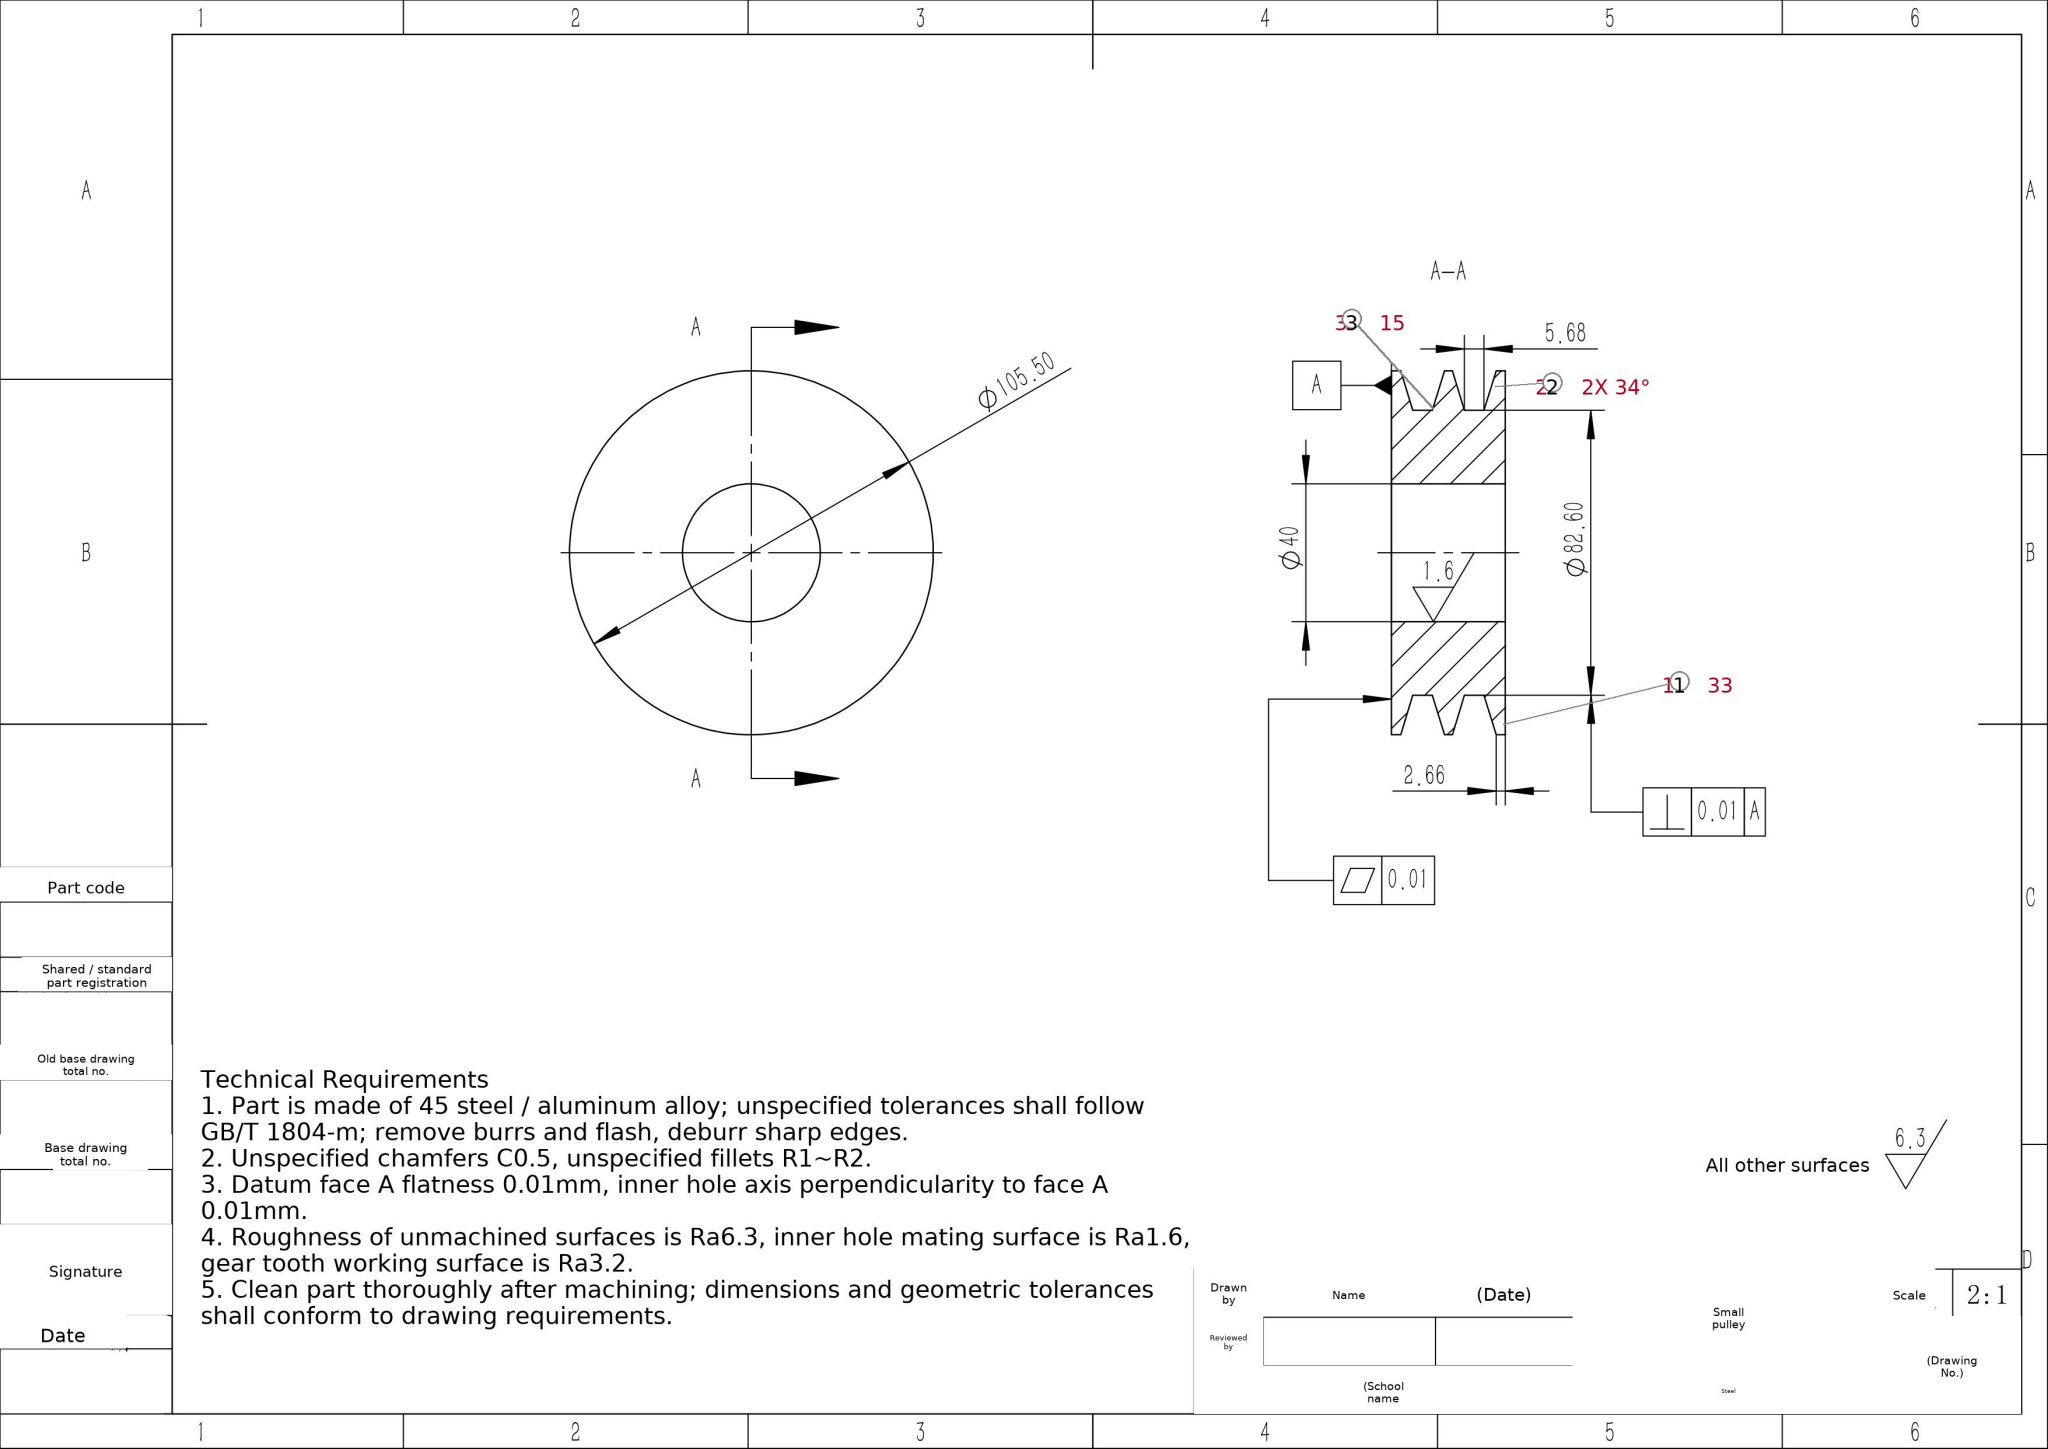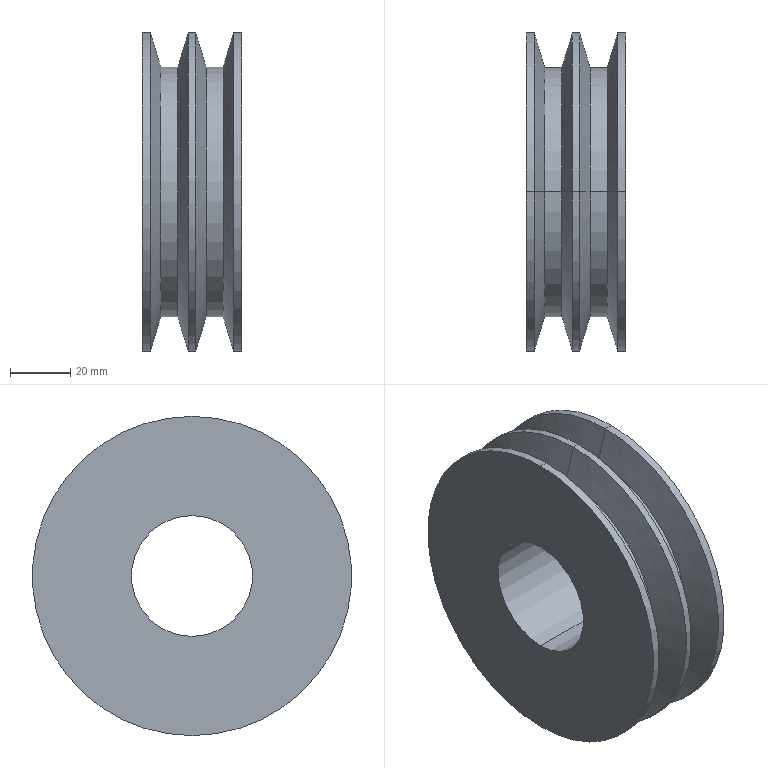Part | SolidWorks | mm | material 45 steel / aluminum alloy | 1 solid | 22 faces | box 33 x 105.5 x 105.5 mm | volume 183925 mm3 | cylinder 12 | cone 8 | plane 2 | commonest cylinder face diameters 105.5 x6 82.6 x4 40 x2
build123d program:
from build123d import *

# Parameters (mm, degrees)
LPATTERN1_COUNT         = 2
LPATTERN1_PITCH         = 15
CHAMFER1_SIZE           = 1
SKETCH4_W               = 5
SKETCH4_H               = 2.3
CUT_EXTRUDE1_DEPTH      = 82.573
CUT_EXTRUDE2_DEPTH      = 82.173
CUT_EXTRUDE2_DEPTH_BACK = 82.173
SKETCH5_R               = 20


with BuildPart() as part:
    # Sketch1 → Revolve1 (revolve)
    with BuildSketch(Plane.XY, mode=Mode.PRIVATE) as revolve1_sk:
        Polygon((0, 8), (0, 52.75), (33, 52.75), (33, 16), (32, 16), (32, 8), align=None)
    revolve(revolve1_sk.sketch.rotate(Axis((0, 0, 0), (1, 0, 0)), 90), axis=Axis((0, 0, 0), (1, 0, 0)))

    # Sketch2 → Cut-Revolve1 (revolve, cut)
    with BuildSketch(Plane.XY, mode=Mode.PRIVATE) as cut_revolve1_sk:
        Polygon((11.84, 41.3), (15.341, 52.75), (2.659, 52.75), (6.16, 41.3), align=None)
    cut_revolve1 = revolve(cut_revolve1_sk.sketch.rotate(Axis((0, 0, 0), (1, 0, 0)), 90), axis=Axis((0, 0, 0), (1, 0, 0)), mode=Mode.SUBTRACT)

    # LPattern1: Cut-Revolve1 ×2
    with Locations(*[(i * LPATTERN1_PITCH, 0, 0) for i in range(1, LPATTERN1_COUNT)]):
        add(cut_revolve1, mode=Mode.SUBTRACT)

    # Chamfer1
    chamfer1_edges = [part.edges().sort_by_distance(p)[0] for p in [
        (0, 0, -8),
        (32, 0, -8),
    ]]
    chamfer(chamfer1_edges, length=CHAMFER1_SIZE)

    # Sketch4 → Cut-Extrude1 (cut, through all)
    with BuildSketch(Plane.ZY):
        with Locations((0, 8.749)):
            Rectangle(SKETCH4_W, SKETCH4_H)
    extrude(amount=-CUT_EXTRUDE1_DEPTH, mode=Mode.SUBTRACT)

    # Sketch5 → Cut-Extrude2 (cut, two sides: drawn at the far end of the back side and taken through both)
    with BuildSketch(Plane(origin=(32, 0, 0), x_dir=(0, 0, -1), z_dir=(1, 0, 0)).offset(-CUT_EXTRUDE2_DEPTH_BACK)):
        Circle(SKETCH5_R)
    extrude(amount=CUT_EXTRUDE2_DEPTH + CUT_EXTRUDE2_DEPTH_BACK, mode=Mode.SUBTRACT)


solid = part.part
STEP:
#1=CARTESIAN_POINT('',(0.,0.,20.));
#2=VERTEX_POINT('',#1);
#3=CARTESIAN_POINT('',(0.,0.,-20.));
#4=VERTEX_POINT('',#3);
#5=CARTESIAN_POINT('',(0.,0.,0.));
#6=DIRECTION('',(1.,0.,0.));
#7=DIRECTION('',(0.,0.,-1.));
#8=AXIS2_PLACEMENT_3D('',#5,#6,#7);
#9=CIRCLE('',#8,20.);
#10=EDGE_CURVE('',#2,#4,#9,.T.);
#11=ORIENTED_EDGE('',*,*,#10,.F.);
#12=CARTESIAN_POINT('',(33.,0.,20.));
#13=VERTEX_POINT('',#12);
#14=CARTESIAN_POINT('',(0.,0.,20.));
#15=DIRECTION('',(1.,0.,0.));
#16=VECTOR('',#15,1000.);
#17=LINE('',#14,#16);
#18=EDGE_CURVE('',#2,#13,#17,.T.);
#19=ORIENTED_EDGE('',*,*,#18,.T.);
#20=CARTESIAN_POINT('',(33.,0.,-20.));
#21=VERTEX_POINT('',#20);
#22=CARTESIAN_POINT('',(33.,0.,0.));
#23=DIRECTION('',(1.,0.,0.));
#24=DIRECTION('',(0.,0.,-1.));
#25=AXIS2_PLACEMENT_3D('',#22,#23,#24);
#26=CIRCLE('',#25,20.);
#27=EDGE_CURVE('',#13,#21,#26,.T.);
#28=ORIENTED_EDGE('',*,*,#27,.T.);
#29=CARTESIAN_POINT('',(0.,0.,-20.));
#30=DIRECTION('',(1.,0.,0.));
#31=VECTOR('',#30,1000.);
#32=LINE('',#29,#31);
#33=EDGE_CURVE('',#4,#21,#32,.T.);
#34=ORIENTED_EDGE('',*,*,#33,.F.);
#35=EDGE_LOOP('',(#11,#19,#28,#34));
#36=FACE_OUTER_BOUND('',#35,.T.);
#37=CARTESIAN_POINT('',(0.,0.,0.));
#38=DIRECTION('',(1.,0.,0.));
#39=DIRECTION('',(0.,0.,-1.));
#40=AXIS2_PLACEMENT_3D('',#37,#38,#39);
#41=CYLINDRICAL_SURFACE('',#40,20.);
#42=ADVANCED_FACE('',(#36),#41,.F.);
#43=CARTESIAN_POINT('',(21.16,0.,41.3));
#44=VERTEX_POINT('',#43);
#45=CARTESIAN_POINT('',(21.16,0.,-41.3));
#46=VERTEX_POINT('',#45);
#47=CARTESIAN_POINT('',(21.16,0.,0.));
#48=DIRECTION('',(-1.,0.,0.));
#49=DIRECTION('',(0.,0.,1.));
#50=AXIS2_PLACEMENT_3D('',#47,#48,#49);
#51=CIRCLE('',#50,41.3);
#52=EDGE_CURVE('',#44,#46,#51,.T.);
#53=ORIENTED_EDGE('',*,*,#52,.T.);
#54=CARTESIAN_POINT('',(17.659,0.,-52.75));
#55=VERTEX_POINT('',#54);
#56=CARTESIAN_POINT('',(17.659,0.,-52.75));
#57=DIRECTION('',(-0.2924,0.,-0.9563));
#58=VECTOR('',#57,1000.);
#59=LINE('',#56,#58);
#60=EDGE_CURVE('',#46,#55,#59,.T.);
#61=ORIENTED_EDGE('',*,*,#60,.T.);
#62=CARTESIAN_POINT('',(17.659,0.,52.75));
#63=VERTEX_POINT('',#62);
#64=CARTESIAN_POINT('',(17.659,0.,0.));
#65=DIRECTION('',(-1.,0.,0.));
#66=DIRECTION('',(0.,0.,1.));
#67=AXIS2_PLACEMENT_3D('',#64,#65,#66);
#68=CIRCLE('',#67,52.75);
#69=EDGE_CURVE('',#63,#55,#68,.T.);
#70=ORIENTED_EDGE('',*,*,#69,.F.);
#71=CARTESIAN_POINT('',(17.659,0.,52.75));
#72=DIRECTION('',(-0.2924,0.,0.9563));
#73=VECTOR('',#72,1000.);
#74=LINE('',#71,#73);
#75=EDGE_CURVE('',#44,#63,#74,.T.);
#76=ORIENTED_EDGE('',*,*,#75,.F.);
#77=EDGE_LOOP('',(#53,#61,#70,#76));
#78=FACE_OUTER_BOUND('',#77,.T.);
#79=CARTESIAN_POINT('',(17.659,0.,0.));
#80=DIRECTION('',(-1.,0.,0.));
#81=DIRECTION('',(0.,0.,1.));
#82=AXIS2_PLACEMENT_3D('',#79,#80,#81);
#83=CONICAL_SURFACE('',#82,52.75,1.274);
#84=ADVANCED_FACE('',(#78),#83,.T.);
#85=CARTESIAN_POINT('',(26.84,0.,41.3));
#86=VERTEX_POINT('',#85);
#87=CARTESIAN_POINT('',(26.84,0.,-41.3));
#88=VERTEX_POINT('',#87);
#89=CARTESIAN_POINT('',(26.84,0.,0.));
#90=DIRECTION('',(-1.,0.,0.));
#91=DIRECTION('',(0.,0.,1.));
#92=AXIS2_PLACEMENT_3D('',#89,#90,#91);
#93=CIRCLE('',#92,41.3);
#94=EDGE_CURVE('',#86,#88,#93,.T.);
#95=ORIENTED_EDGE('',*,*,#94,.F.);
#96=CARTESIAN_POINT('',(30.341,0.,52.75));
#97=VERTEX_POINT('',#96);
#98=CARTESIAN_POINT('',(26.84,0.,41.3));
#99=DIRECTION('',(0.2924,0.,0.9563));
#100=VECTOR('',#99,1000.);
#101=LINE('',#98,#100);
#102=EDGE_CURVE('',#86,#97,#101,.T.);
#103=ORIENTED_EDGE('',*,*,#102,.T.);
#104=CARTESIAN_POINT('',(30.341,0.,-52.75));
#105=VERTEX_POINT('',#104);
#106=CARTESIAN_POINT('',(30.341,0.,0.));
#107=DIRECTION('',(-1.,0.,0.));
#108=DIRECTION('',(0.,0.,1.));
#109=AXIS2_PLACEMENT_3D('',#106,#107,#108);
#110=CIRCLE('',#109,52.75);
#111=EDGE_CURVE('',#97,#105,#110,.T.);
#112=ORIENTED_EDGE('',*,*,#111,.T.);
#113=CARTESIAN_POINT('',(26.84,0.,-41.3));
#114=DIRECTION('',(0.2924,0.,-0.9563));
#115=VECTOR('',#114,1000.);
#116=LINE('',#113,#115);
#117=EDGE_CURVE('',#88,#105,#116,.T.);
#118=ORIENTED_EDGE('',*,*,#117,.F.);
#119=EDGE_LOOP('',(#95,#103,#112,#118));
#120=FACE_OUTER_BOUND('',#119,.T.);
#121=CARTESIAN_POINT('',(26.84,0.,0.));
#122=DIRECTION('',(1.,0.,0.));
#123=DIRECTION('',(0.,0.,-1.));
#124=AXIS2_PLACEMENT_3D('',#121,#122,#123);
#125=CONICAL_SURFACE('',#124,41.3,1.274);
#126=ADVANCED_FACE('',(#120),#125,.T.);
#127=ORIENTED_EDGE('',*,*,#94,.T.);
#128=CARTESIAN_POINT('',(15.,0.,-41.3));
#129=DIRECTION('',(-1.,0.,0.));
#130=VECTOR('',#129,1000.);
#131=LINE('',#128,#130);
#132=EDGE_CURVE('',#88,#46,#131,.T.);
#133=ORIENTED_EDGE('',*,*,#132,.T.);
#134=ORIENTED_EDGE('',*,*,#52,.F.);
#135=CARTESIAN_POINT('',(15.,0.,41.3));
#136=DIRECTION('',(-1.,0.,0.));
#137=VECTOR('',#136,1000.);
#138=LINE('',#135,#137);
#139=EDGE_CURVE('',#86,#44,#138,.T.);
#140=ORIENTED_EDGE('',*,*,#139,.F.);
#141=EDGE_LOOP('',(#127,#133,#134,#140));
#142=FACE_OUTER_BOUND('',#141,.T.);
#143=CARTESIAN_POINT('',(15.,0.,0.));
#144=DIRECTION('',(-1.,0.,0.));
#145=DIRECTION('',(0.,0.,1.));
#146=AXIS2_PLACEMENT_3D('',#143,#144,#145);
#147=CYLINDRICAL_SURFACE('',#146,41.3);
#148=ADVANCED_FACE('',(#142),#147,.T.);
#149=CARTESIAN_POINT('',(6.16,0.,41.3));
#150=VERTEX_POINT('',#149);
#151=CARTESIAN_POINT('',(6.16,0.,-41.3));
#152=VERTEX_POINT('',#151);
#153=CARTESIAN_POINT('',(6.16,0.,0.));
#154=DIRECTION('',(-1.,0.,0.));
#155=DIRECTION('',(0.,0.,1.));
#156=AXIS2_PLACEMENT_3D('',#153,#154,#155);
#157=CIRCLE('',#156,41.3);
#158=EDGE_CURVE('',#150,#152,#157,.T.);
#159=ORIENTED_EDGE('',*,*,#158,.T.);
#160=CARTESIAN_POINT('',(2.659,0.,-52.75));
#161=VERTEX_POINT('',#160);
#162=CARTESIAN_POINT('',(2.659,0.,-52.75));
#163=DIRECTION('',(-0.2924,0.,-0.9563));
#164=VECTOR('',#163,1000.);
#165=LINE('',#162,#164);
#166=EDGE_CURVE('',#152,#161,#165,.T.);
#167=ORIENTED_EDGE('',*,*,#166,.T.);
#168=CARTESIAN_POINT('',(2.659,0.,52.75));
#169=VERTEX_POINT('',#168);
#170=CARTESIAN_POINT('',(2.659,0.,0.));
#171=DIRECTION('',(-1.,0.,0.));
#172=DIRECTION('',(0.,0.,1.));
#173=AXIS2_PLACEMENT_3D('',#170,#171,#172);
#174=CIRCLE('',#173,52.75);
#175=EDGE_CURVE('',#169,#161,#174,.T.);
#176=ORIENTED_EDGE('',*,*,#175,.F.);
#177=CARTESIAN_POINT('',(2.659,0.,52.75));
#178=DIRECTION('',(-0.2924,0.,0.9563));
#179=VECTOR('',#178,1000.);
#180=LINE('',#177,#179);
#181=EDGE_CURVE('',#150,#169,#180,.T.);
#182=ORIENTED_EDGE('',*,*,#181,.F.);
#183=EDGE_LOOP('',(#159,#167,#176,#182));
#184=FACE_OUTER_BOUND('',#183,.T.);
#185=CARTESIAN_POINT('',(2.659,0.,0.));
#186=DIRECTION('',(-1.,0.,0.));
#187=DIRECTION('',(0.,0.,1.));
#188=AXIS2_PLACEMENT_3D('',#185,#186,#187);
#189=CONICAL_SURFACE('',#188,52.75,1.274);
#190=ADVANCED_FACE('',(#184),#189,.T.);
#191=CARTESIAN_POINT('',(11.84,0.,41.3));
#192=VERTEX_POINT('',#191);
#193=CARTESIAN_POINT('',(11.84,0.,-41.3));
#194=VERTEX_POINT('',#193);
#195=CARTESIAN_POINT('',(11.84,0.,0.));
#196=DIRECTION('',(-1.,0.,0.));
#197=DIRECTION('',(0.,0.,1.));
#198=AXIS2_PLACEMENT_3D('',#195,#196,#197);
#199=CIRCLE('',#198,41.3);
#200=EDGE_CURVE('',#192,#194,#199,.T.);
#201=ORIENTED_EDGE('',*,*,#200,.F.);
#202=CARTESIAN_POINT('',(15.341,0.,52.75));
#203=VERTEX_POINT('',#202);
#204=CARTESIAN_POINT('',(11.84,0.,41.3));
#205=DIRECTION('',(0.2924,0.,0.9563));
#206=VECTOR('',#205,1000.);
#207=LINE('',#204,#206);
#208=EDGE_CURVE('',#192,#203,#207,.T.);
#209=ORIENTED_EDGE('',*,*,#208,.T.);
#210=CARTESIAN_POINT('',(15.341,0.,-52.75));
#211=VERTEX_POINT('',#210);
#212=CARTESIAN_POINT('',(15.341,0.,0.));
#213=DIRECTION('',(-1.,0.,0.));
#214=DIRECTION('',(0.,0.,1.));
#215=AXIS2_PLACEMENT_3D('',#212,#213,#214);
#216=CIRCLE('',#215,52.75);
#217=EDGE_CURVE('',#203,#211,#216,.T.);
#218=ORIENTED_EDGE('',*,*,#217,.T.);
#219=CARTESIAN_POINT('',(11.84,0.,-41.3));
#220=DIRECTION('',(0.2924,0.,-0.9563));
#221=VECTOR('',#220,1000.);
#222=LINE('',#219,#221);
#223=EDGE_CURVE('',#194,#211,#222,.T.);
#224=ORIENTED_EDGE('',*,*,#223,.F.);
#225=EDGE_LOOP('',(#201,#209,#218,#224));
#226=FACE_OUTER_BOUND('',#225,.T.);
#227=CARTESIAN_POINT('',(11.84,0.,0.));
#228=DIRECTION('',(1.,0.,0.));
#229=DIRECTION('',(0.,0.,-1.));
#230=AXIS2_PLACEMENT_3D('',#227,#228,#229);
#231=CONICAL_SURFACE('',#230,41.3,1.274);
#232=ADVANCED_FACE('',(#226),#231,.T.);
#233=ORIENTED_EDGE('',*,*,#200,.T.);
#234=CARTESIAN_POINT('',(0.,0.,-41.3));
#235=DIRECTION('',(-1.,0.,0.));
#236=VECTOR('',#235,1000.);
#237=LINE('',#234,#236);
#238=EDGE_CURVE('',#194,#152,#237,.T.);
#239=ORIENTED_EDGE('',*,*,#238,.T.);
#240=ORIENTED_EDGE('',*,*,#158,.F.);
#241=CARTESIAN_POINT('',(0.,0.,41.3));
#242=DIRECTION('',(-1.,0.,0.));
#243=VECTOR('',#242,1000.);
#244=LINE('',#241,#243);
#245=EDGE_CURVE('',#192,#150,#244,.T.);
#246=ORIENTED_EDGE('',*,*,#245,.F.);
#247=EDGE_LOOP('',(#233,#239,#240,#246));
#248=FACE_OUTER_BOUND('',#247,.T.);
#249=CARTESIAN_POINT('',(0.,0.,0.));
#250=DIRECTION('',(-1.,0.,0.));
#251=DIRECTION('',(0.,0.,1.));
#252=AXIS2_PLACEMENT_3D('',#249,#250,#251);
#253=CYLINDRICAL_SURFACE('',#252,41.3);
#254=ADVANCED_FACE('',(#248),#253,.T.);
#255=ORIENTED_EDGE('',*,*,#175,.T.);
#256=CARTESIAN_POINT('',(0.,0.,-52.75));
#257=VERTEX_POINT('',#256);
#258=CARTESIAN_POINT('',(0.,0.,-52.75));
#259=DIRECTION('',(-1.,0.,0.));
#260=VECTOR('',#259,1000.);
#261=LINE('',#258,#260);
#262=EDGE_CURVE('',#161,#257,#261,.T.);
#263=ORIENTED_EDGE('',*,*,#262,.T.);
#264=CARTESIAN_POINT('',(0.,0.,52.75));
#265=VERTEX_POINT('',#264);
#266=CARTESIAN_POINT('',(0.,0.,0.));
#267=DIRECTION('',(-1.,0.,0.));
#268=DIRECTION('',(0.,0.,1.));
#269=AXIS2_PLACEMENT_3D('',#266,#267,#268);
#270=CIRCLE('',#269,52.75);
#271=EDGE_CURVE('',#265,#257,#270,.T.);
#272=ORIENTED_EDGE('',*,*,#271,.F.);
#273=CARTESIAN_POINT('',(0.,0.,52.75));
#274=DIRECTION('',(-1.,0.,0.));
#275=VECTOR('',#274,1000.);
#276=LINE('',#273,#275);
#277=EDGE_CURVE('',#169,#265,#276,.T.);
#278=ORIENTED_EDGE('',*,*,#277,.F.);
#279=EDGE_LOOP('',(#255,#263,#272,#278));
#280=FACE_OUTER_BOUND('',#279,.T.);
#281=CARTESIAN_POINT('',(0.,0.,0.));
#282=DIRECTION('',(-1.,0.,0.));
#283=DIRECTION('',(0.,0.,1.));
#284=AXIS2_PLACEMENT_3D('',#281,#282,#283);
#285=CYLINDRICAL_SURFACE('',#284,52.75);
#286=ADVANCED_FACE('',(#280),#285,.T.);
#287=ORIENTED_EDGE('',*,*,#69,.T.);
#288=CARTESIAN_POINT('',(0.,0.,-52.75));
#289=DIRECTION('',(-1.,0.,0.));
#290=VECTOR('',#289,1000.);
#291=LINE('',#288,#290);
#292=EDGE_CURVE('',#55,#211,#291,.T.);
#293=ORIENTED_EDGE('',*,*,#292,.T.);
#294=ORIENTED_EDGE('',*,*,#217,.F.);
#295=CARTESIAN_POINT('',(0.,0.,52.75));
#296=DIRECTION('',(-1.,0.,0.));
#297=VECTOR('',#296,1000.);
#298=LINE('',#295,#297);
#299=EDGE_CURVE('',#63,#203,#298,.T.);
#300=ORIENTED_EDGE('',*,*,#299,.F.);
#301=EDGE_LOOP('',(#287,#293,#294,#300));
#302=FACE_OUTER_BOUND('',#301,.T.);
#303=CARTESIAN_POINT('',(0.,0.,0.));
#304=DIRECTION('',(-1.,0.,0.));
#305=DIRECTION('',(0.,0.,1.));
#306=AXIS2_PLACEMENT_3D('',#303,#304,#305);
#307=CYLINDRICAL_SURFACE('',#306,52.75);
#308=ADVANCED_FACE('',(#302),#307,.T.);
#309=CARTESIAN_POINT('',(33.,0.,52.75));
#310=VERTEX_POINT('',#309);
#311=CARTESIAN_POINT('',(33.,0.,-52.75));
#312=VERTEX_POINT('',#311);
#313=CARTESIAN_POINT('',(33.,0.,0.));
#314=DIRECTION('',(-1.,0.,0.));
#315=DIRECTION('',(0.,0.,1.));
#316=AXIS2_PLACEMENT_3D('',#313,#314,#315);
#317=CIRCLE('',#316,52.75);
#318=EDGE_CURVE('',#310,#312,#317,.T.);
#319=ORIENTED_EDGE('',*,*,#318,.T.);
#320=CARTESIAN_POINT('',(0.,0.,-52.75));
#321=DIRECTION('',(-1.,0.,0.));
#322=VECTOR('',#321,1000.);
#323=LINE('',#320,#322);
#324=EDGE_CURVE('',#312,#105,#323,.T.);
#325=ORIENTED_EDGE('',*,*,#324,.T.);
#326=ORIENTED_EDGE('',*,*,#111,.F.);
#327=CARTESIAN_POINT('',(0.,0.,52.75));
#328=DIRECTION('',(-1.,0.,0.));
#329=VECTOR('',#328,1000.);
#330=LINE('',#327,#329);
#331=EDGE_CURVE('',#310,#97,#330,.T.);
#332=ORIENTED_EDGE('',*,*,#331,.F.);
#333=EDGE_LOOP('',(#319,#325,#326,#332));
#334=FACE_OUTER_BOUND('',#333,.T.);
#335=CARTESIAN_POINT('',(0.,0.,0.));
#336=DIRECTION('',(-1.,0.,0.));
#337=DIRECTION('',(0.,0.,1.));
#338=AXIS2_PLACEMENT_3D('',#335,#336,#337);
#339=CYLINDRICAL_SURFACE('',#338,52.75);
#340=ADVANCED_FACE('',(#334),#339,.T.);
#341=ORIENTED_EDGE('',*,*,#324,.F.);
#342=CARTESIAN_POINT('',(33.,0.,0.));
#343=DIRECTION('',(-1.,0.,0.));
#344=DIRECTION('',(0.,0.,1.));
#345=AXIS2_PLACEMENT_3D('',#342,#343,#344);
#346=CIRCLE('',#345,52.75);
#347=EDGE_CURVE('',#312,#310,#346,.T.);
#348=ORIENTED_EDGE('',*,*,#347,.T.);
#349=ORIENTED_EDGE('',*,*,#331,.T.);
#350=CARTESIAN_POINT('',(30.341,0.,0.));
#351=DIRECTION('',(-1.,0.,0.));
#352=DIRECTION('',(0.,0.,1.));
#353=AXIS2_PLACEMENT_3D('',#350,#351,#352);
#354=CIRCLE('',#353,52.75);
#355=EDGE_CURVE('',#105,#97,#354,.T.);
#356=ORIENTED_EDGE('',*,*,#355,.F.);
#357=EDGE_LOOP('',(#341,#348,#349,#356));
#358=FACE_OUTER_BOUND('',#357,.T.);
#359=CARTESIAN_POINT('',(0.,0.,0.));
#360=DIRECTION('',(-1.,0.,0.));
#361=DIRECTION('',(0.,0.,1.));
#362=AXIS2_PLACEMENT_3D('',#359,#360,#361);
#363=CYLINDRICAL_SURFACE('',#362,52.75);
#364=ADVANCED_FACE('',(#358),#363,.T.);
#365=ORIENTED_EDGE('',*,*,#292,.F.);
#366=CARTESIAN_POINT('',(17.659,0.,0.));
#367=DIRECTION('',(-1.,0.,0.));
#368=DIRECTION('',(0.,0.,1.));
#369=AXIS2_PLACEMENT_3D('',#366,#367,#368);
#370=CIRCLE('',#369,52.75);
#371=EDGE_CURVE('',#55,#63,#370,.T.);
#372=ORIENTED_EDGE('',*,*,#371,.T.);
#373=ORIENTED_EDGE('',*,*,#299,.T.);
#374=CARTESIAN_POINT('',(15.341,0.,0.));
#375=DIRECTION('',(-1.,0.,0.));
#376=DIRECTION('',(0.,0.,1.));
#377=AXIS2_PLACEMENT_3D('',#374,#375,#376);
#378=CIRCLE('',#377,52.75);
#379=EDGE_CURVE('',#211,#203,#378,.T.);
#380=ORIENTED_EDGE('',*,*,#379,.F.);
#381=EDGE_LOOP('',(#365,#372,#373,#380));
#382=FACE_OUTER_BOUND('',#381,.T.);
#383=CARTESIAN_POINT('',(0.,0.,0.));
#384=DIRECTION('',(-1.,0.,0.));
#385=DIRECTION('',(0.,0.,1.));
#386=AXIS2_PLACEMENT_3D('',#383,#384,#385);
#387=CYLINDRICAL_SURFACE('',#386,52.75);
#388=ADVANCED_FACE('',(#382),#387,.T.);
#389=ORIENTED_EDGE('',*,*,#262,.F.);
#390=CARTESIAN_POINT('',(2.659,0.,0.));
#391=DIRECTION('',(-1.,0.,0.));
#392=DIRECTION('',(0.,0.,1.));
#393=AXIS2_PLACEMENT_3D('',#390,#391,#392);
#394=CIRCLE('',#393,52.75);
#395=EDGE_CURVE('',#161,#169,#394,.T.);
#396=ORIENTED_EDGE('',*,*,#395,.T.);
#397=ORIENTED_EDGE('',*,*,#277,.T.);
#398=CARTESIAN_POINT('',(0.,0.,0.));
#399=DIRECTION('',(-1.,0.,0.));
#400=DIRECTION('',(0.,0.,1.));
#401=AXIS2_PLACEMENT_3D('',#398,#399,#400);
#402=CIRCLE('',#401,52.75);
#403=EDGE_CURVE('',#257,#265,#402,.T.);
#404=ORIENTED_EDGE('',*,*,#403,.F.);
#405=EDGE_LOOP('',(#389,#396,#397,#404));
#406=FACE_OUTER_BOUND('',#405,.T.);
#407=CARTESIAN_POINT('',(0.,0.,0.));
#408=DIRECTION('',(-1.,0.,0.));
#409=DIRECTION('',(0.,0.,1.));
#410=AXIS2_PLACEMENT_3D('',#407,#408,#409);
#411=CYLINDRICAL_SURFACE('',#410,52.75);
#412=ADVANCED_FACE('',(#406),#411,.T.);
#413=CARTESIAN_POINT('',(33.,0.,0.));
#414=DIRECTION('',(1.,0.,0.));
#415=DIRECTION('',(0.,0.,-1.));
#416=AXIS2_PLACEMENT_3D('',#413,#414,#415);
#417=CIRCLE('',#416,20.);
#418=EDGE_CURVE('',#21,#13,#417,.T.);
#419=ORIENTED_EDGE('',*,*,#418,.F.);
#420=ORIENTED_EDGE('',*,*,#27,.F.);
#421=EDGE_LOOP('',(#419,#420));
#422=FACE_BOUND('',#421,.T.);
#423=ORIENTED_EDGE('',*,*,#318,.F.);
#424=ORIENTED_EDGE('',*,*,#347,.F.);
#425=EDGE_LOOP('',(#423,#424));
#426=FACE_OUTER_BOUND('',#425,.T.);
#427=CARTESIAN_POINT('',(33.,52.75,0.));
#428=DIRECTION('',(-1.,0.,0.));
#429=DIRECTION('',(0.,0.,1.));
#430=AXIS2_PLACEMENT_3D('',#427,#428,#429);
#431=PLANE('',#430);
#432=ADVANCED_FACE('',(#422,#426),#431,.F.);
#433=CARTESIAN_POINT('',(0.,0.,0.));
#434=DIRECTION('',(1.,0.,0.));
#435=DIRECTION('',(0.,0.,-1.));
#436=AXIS2_PLACEMENT_3D('',#433,#434,#435);
#437=CIRCLE('',#436,20.);
#438=EDGE_CURVE('',#4,#2,#437,.T.);
#439=ORIENTED_EDGE('',*,*,#438,.T.);
#440=ORIENTED_EDGE('',*,*,#10,.T.);
#441=EDGE_LOOP('',(#439,#440));
#442=FACE_BOUND('',#441,.T.);
#443=ORIENTED_EDGE('',*,*,#271,.T.);
#444=ORIENTED_EDGE('',*,*,#403,.T.);
#445=EDGE_LOOP('',(#443,#444));
#446=FACE_OUTER_BOUND('',#445,.T.);
#447=CARTESIAN_POINT('',(0.,8.,0.));
#448=DIRECTION('',(1.,0.,0.));
#449=DIRECTION('',(0.,0.,-1.));
#450=AXIS2_PLACEMENT_3D('',#447,#448,#449);
#451=PLANE('',#450);
#452=ADVANCED_FACE('',(#442,#446),#451,.F.);
#453=ORIENTED_EDGE('',*,*,#238,.F.);
#454=CARTESIAN_POINT('',(11.84,0.,0.));
#455=DIRECTION('',(-1.,0.,0.));
#456=DIRECTION('',(0.,0.,1.));
#457=AXIS2_PLACEMENT_3D('',#454,#455,#456);
#458=CIRCLE('',#457,41.3);
#459=EDGE_CURVE('',#194,#192,#458,.T.);
#460=ORIENTED_EDGE('',*,*,#459,.T.);
#461=ORIENTED_EDGE('',*,*,#245,.T.);
#462=CARTESIAN_POINT('',(6.16,0.,0.));
#463=DIRECTION('',(-1.,0.,0.));
#464=DIRECTION('',(0.,0.,1.));
#465=AXIS2_PLACEMENT_3D('',#462,#463,#464);
#466=CIRCLE('',#465,41.3);
#467=EDGE_CURVE('',#152,#150,#466,.T.);
#468=ORIENTED_EDGE('',*,*,#467,.F.);
#469=EDGE_LOOP('',(#453,#460,#461,#468));
#470=FACE_OUTER_BOUND('',#469,.T.);
#471=CARTESIAN_POINT('',(0.,0.,0.));
#472=DIRECTION('',(-1.,0.,0.));
#473=DIRECTION('',(0.,0.,1.));
#474=AXIS2_PLACEMENT_3D('',#471,#472,#473);
#475=CYLINDRICAL_SURFACE('',#474,41.3);
#476=ADVANCED_FACE('',(#470),#475,.T.);
#477=ORIENTED_EDGE('',*,*,#208,.F.);
#478=ORIENTED_EDGE('',*,*,#459,.F.);
#479=ORIENTED_EDGE('',*,*,#223,.T.);
#480=ORIENTED_EDGE('',*,*,#379,.T.);
#481=EDGE_LOOP('',(#477,#478,#479,#480));
#482=FACE_OUTER_BOUND('',#481,.T.);
#483=CARTESIAN_POINT('',(11.84,0.,0.));
#484=DIRECTION('',(1.,0.,0.));
#485=DIRECTION('',(0.,0.,-1.));
#486=AXIS2_PLACEMENT_3D('',#483,#484,#485);
#487=CONICAL_SURFACE('',#486,41.3,1.274);
#488=ADVANCED_FACE('',(#482),#487,.T.);
#489=ORIENTED_EDGE('',*,*,#166,.F.);
#490=ORIENTED_EDGE('',*,*,#467,.T.);
#491=ORIENTED_EDGE('',*,*,#181,.T.);
#492=ORIENTED_EDGE('',*,*,#395,.F.);
#493=EDGE_LOOP('',(#489,#490,#491,#492));
#494=FACE_OUTER_BOUND('',#493,.T.);
#495=CARTESIAN_POINT('',(2.659,0.,0.));
#496=DIRECTION('',(-1.,0.,0.));
#497=DIRECTION('',(0.,0.,1.));
#498=AXIS2_PLACEMENT_3D('',#495,#496,#497);
#499=CONICAL_SURFACE('',#498,52.75,1.274);
#500=ADVANCED_FACE('',(#494),#499,.T.);
#501=ORIENTED_EDGE('',*,*,#132,.F.);
#502=CARTESIAN_POINT('',(26.84,0.,0.));
#503=DIRECTION('',(-1.,0.,0.));
#504=DIRECTION('',(0.,0.,1.));
#505=AXIS2_PLACEMENT_3D('',#502,#503,#504);
#506=CIRCLE('',#505,41.3);
#507=EDGE_CURVE('',#88,#86,#506,.T.);
#508=ORIENTED_EDGE('',*,*,#507,.T.);
#509=ORIENTED_EDGE('',*,*,#139,.T.);
#510=CARTESIAN_POINT('',(21.16,0.,0.));
#511=DIRECTION('',(-1.,0.,0.));
#512=DIRECTION('',(0.,0.,1.));
#513=AXIS2_PLACEMENT_3D('',#510,#511,#512);
#514=CIRCLE('',#513,41.3);
#515=EDGE_CURVE('',#46,#44,#514,.T.);
#516=ORIENTED_EDGE('',*,*,#515,.F.);
#517=EDGE_LOOP('',(#501,#508,#509,#516));
#518=FACE_OUTER_BOUND('',#517,.T.);
#519=CARTESIAN_POINT('',(15.,0.,0.));
#520=DIRECTION('',(-1.,0.,0.));
#521=DIRECTION('',(0.,0.,1.));
#522=AXIS2_PLACEMENT_3D('',#519,#520,#521);
#523=CYLINDRICAL_SURFACE('',#522,41.3);
#524=ADVANCED_FACE('',(#518),#523,.T.);
#525=ORIENTED_EDGE('',*,*,#102,.F.);
#526=ORIENTED_EDGE('',*,*,#507,.F.);
#527=ORIENTED_EDGE('',*,*,#117,.T.);
#528=ORIENTED_EDGE('',*,*,#355,.T.);
#529=EDGE_LOOP('',(#525,#526,#527,#528));
#530=FACE_OUTER_BOUND('',#529,.T.);
#531=CARTESIAN_POINT('',(26.84,0.,0.));
#532=DIRECTION('',(1.,0.,0.));
#533=DIRECTION('',(0.,0.,-1.));
#534=AXIS2_PLACEMENT_3D('',#531,#532,#533);
#535=CONICAL_SURFACE('',#534,41.3,1.274);
#536=ADVANCED_FACE('',(#530),#535,.T.);
#537=ORIENTED_EDGE('',*,*,#60,.F.);
#538=ORIENTED_EDGE('',*,*,#515,.T.);
#539=ORIENTED_EDGE('',*,*,#75,.T.);
#540=ORIENTED_EDGE('',*,*,#371,.F.);
#541=EDGE_LOOP('',(#537,#538,#539,#540));
#542=FACE_OUTER_BOUND('',#541,.T.);
#543=CARTESIAN_POINT('',(17.659,0.,0.));
#544=DIRECTION('',(-1.,0.,0.));
#545=DIRECTION('',(0.,0.,1.));
#546=AXIS2_PLACEMENT_3D('',#543,#544,#545);
#547=CONICAL_SURFACE('',#546,52.75,1.274);
#548=ADVANCED_FACE('',(#542),#547,.T.);
#549=ORIENTED_EDGE('',*,*,#18,.F.);
#550=ORIENTED_EDGE('',*,*,#438,.F.);
#551=ORIENTED_EDGE('',*,*,#33,.T.);
#552=ORIENTED_EDGE('',*,*,#418,.T.);
#553=EDGE_LOOP('',(#549,#550,#551,#552));
#554=FACE_OUTER_BOUND('',#553,.T.);
#555=CARTESIAN_POINT('',(0.,0.,0.));
#556=DIRECTION('',(1.,0.,0.));
#557=DIRECTION('',(0.,0.,-1.));
#558=AXIS2_PLACEMENT_3D('',#555,#556,#557);
#559=CYLINDRICAL_SURFACE('',#558,20.);
#560=ADVANCED_FACE('',(#554),#559,.F.);
#561=CLOSED_SHELL('',(#42,#84,#126,#148,#190,#232,#254,#286,#308,#340,#364,#388,#412,#432,#452,#476,#488,#500,#524,#536,#548,#560));
#562=MANIFOLD_SOLID_BREP('',#561);
#563=CARTESIAN_POINT('',(0.,0.,0.));
#564=DIRECTION('',(0.,0.,1.));
#565=DIRECTION('',(1.,0.,0.));
#566=AXIS2_PLACEMENT_3D('',#563,#564,#565);
#567=(LENGTH_UNIT()NAMED_UNIT(*)SI_UNIT(.MILLI.,.METRE.));
#568=UNCERTAINTY_MEASURE_WITH_UNIT(LENGTH_MEASURE(0.00001),#567,'','');
#569=(NAMED_UNIT(*)PLANE_ANGLE_UNIT()SI_UNIT($,.RADIAN.));
#570=(NAMED_UNIT(*)SI_UNIT($,.STERADIAN.)SOLID_ANGLE_UNIT());
#571=(GEOMETRIC_REPRESENTATION_CONTEXT(3)GLOBAL_UNCERTAINTY_ASSIGNED_CONTEXT((#568))GLOBAL_UNIT_ASSIGNED_CONTEXT((#567,#569,#570))REPRESENTATION_CONTEXT('',''));
#572=ADVANCED_BREP_SHAPE_REPRESENTATION('',(#562,#566),#571);